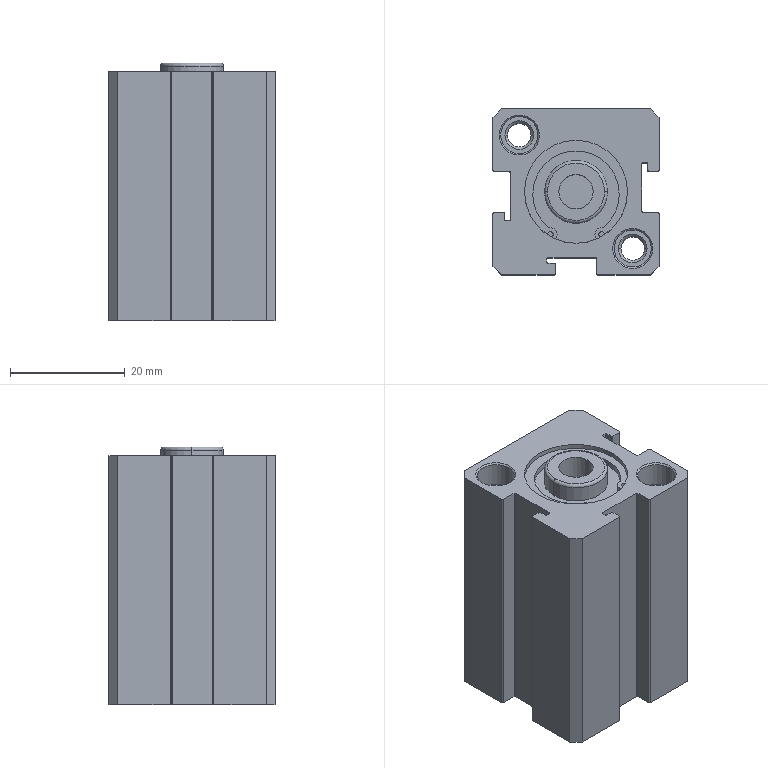Component | SolidWorks | SDA_16x25_0-1_SDA_16x2525_b-1 | 1 solid | 119 faces | volume 25076 mm3 | cylinder 56 | plane 41 | cone 20 | torus 2 | commonest cylinder face diameters 0.4 x18 1 x8 4.134 x8 6.5 x8 15.1 x3 2.4 x3 6 x2 16 x2